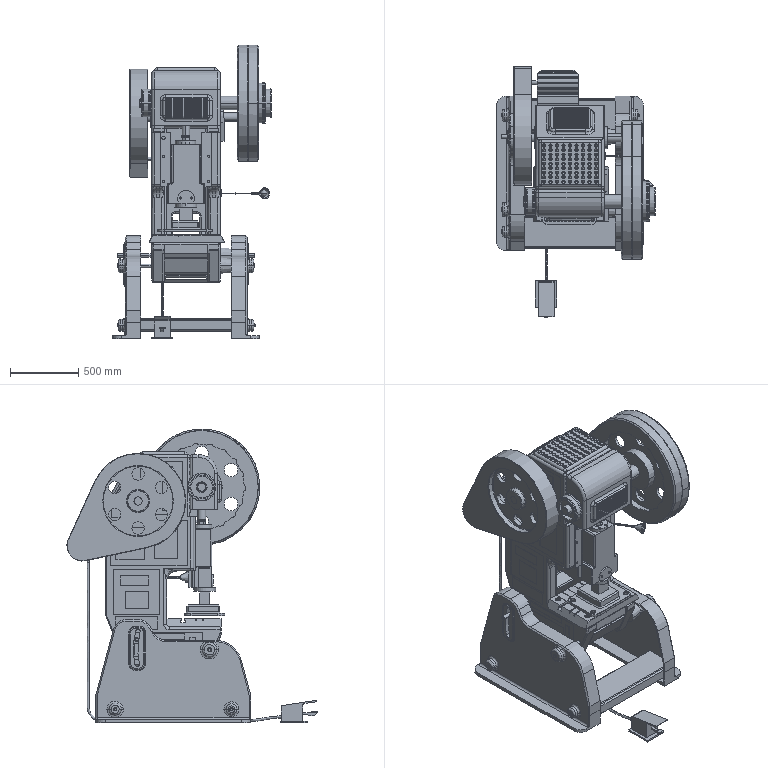Assembly | SolidWorks | mm | 53 component files | 53 solids | 4337 faces | box 1159 x 1828.89 x 2148.9 mm | volume 424193387 mm3 | plane 1614 | cylinder 1553 | cone 588 | spline 500 | torus 65 | sphere 17 | commonest cylinder face diameters 3.8 x373 21.383 x162 789.22 x156 20 x86 40 x68 10 x60 30 x44 61.909 x42
Bill of materials:
AxisHead | 1 |  | Short disc/wheel body with a shallow circumferential groove between two rim flanges, a smaller coaxial cylindrical boss with rounded edge on one face, and a shallow circular recess with a raised lip on the opposite face.
Belt | 3 |  | Thin closed loop shaped like a teardrop / rounded triangle: a large circular arc joined by two straight segments that meet at a small rounded corner. The section is very thin and the loop lies flat in one plane.
Cam | 1 |  | Rectangular block with rounded vertical edges and one large cylindrical through-hole passing through a pair of opposite side faces.
CamAxis | 1 |  | Plain solid cylindrical rod with flat ends.
ConnectingBeam | 2 |  | Elongated rectangular bar with angled chamfers at the end corners, light edge chamfers along the long edges, and a small coaxial cylindrical pin projecting from the centre of each end face. A small circular ring feature sits at the centre of one large face.
ConnectingBlock | 1 |  | Solid rectangular block with filleted or rounded edges on all sides. No holes or other features are visible.
ConnectingRod | 1 |  | Stepped turned pin: a cylindrical shank with a chamfered top and a narrow circumferential groove near its lower end, a hexagonal section below, and a two-step circular flange at the base.
CountersunkScrew | 6 |  | Countersunk (conical) flat-head fastener-like body with a cross-shaped recess in the head, a short reduced-diameter neck under the head, and a longer, larger-diameter cylindrical shank.
CylindricalHeadHexSocketScrew | 4 |  | Cylindrical head with a hexagonal socket on a plain, smaller-diameter cylindrical shank, similar in form to a socket head cap screw.
DriveShaft | 1 |  | Stepped cylinder: a larger-diameter main body with a small axial bore in one end face, and a smaller coaxial cylindrical pin projecting from the other end.
EndCapCover | 1 |  | Flanged circular cap: a thin round flange with six evenly spaced small holes around its edge, and a raised, closed cylindrical boss in the centre with a rounded top edge.
EndFacePressurePlate | 1 |  | Square flat plate of moderate thickness with seven through-holes of at least two diameters in an irregular pattern.
FixedAxis | 2 |  | Short prismatic body with an irregular five-sided, round-cornered cross-section, pierced axially by a straight slender cylindrical rod that sticks out a long way on both ends.
Flywheel | 1 |  | Thick annular ring (short hollow cylinder) with one central through bore and lightly rounded outer edges.
FootSwitch | 1 |  | Long thin wire or rod with a radiused bend, ending in a small box-shaped block with flanges and slots at one end.
Frame | 1 |  | Complex hollow housing or bracket body: a rectangular tube-like upper section with a square through opening, a ribbed raised pad on one face, a side profile with a C-shaped notch and angled lower edge, and an open lower frame.
Gland | 1 |  | Flat circular annular plate with a large central bore and six round through holes evenly spaced on a circle between bore and rim.
GuidePlate | 1 |  | Rectangular bar with a V-shaped groove along one long face and two small round through holes along its length.
LargeGear | 1 |  | Large spur-style gear with many fine straight teeth, a recessed web with six round lightening holes, and a protruding cylindrical hub on one side with a central bore.
LargePulley | 1 |  | Disk-shaped wheel with several circumferential grooves on its outer rim, a recessed face, six round holes on a circle, and a small central hole.
LeftBase | 1 |  | Flat profiled side plate with sloped sides and a raised rounded hump at one upper corner. It has a perimeter lip, a bottom flange along one edge, a curved arc-shaped slot with a raised boss around it, small holes, and cylindrical bosses on the back.
LeftGuideRail | 1 |  | Rectangular bar with a V-shaped groove along one long face and three small round through holes evenly spaced along its length.
Light | 1 |  | Circular disk base with a slender curved rod (S-bend) running to a conical cup-shaped head that holds a sphere.
Motor | 1 |  | Extruded block whose constant cross-section combines a large round lobe with many small radial fins, a rectangular tab with a C-shaped slot, and two rounded notches. It has longitudinal surface grooves, and a small stud with circumferential ribs on a narrow neck sticks out from one end face.
Pinion | 1 |  | Straight-toothed spur gear: a cylindrical body that is fairly wide relative to its diameter, with a central round bore that has one keyway notch.
Plate | 1 |  | Very thin, flat circular disc with no visible holes or features.
PressureBlock | 1 |  | Prismatic block with a rounded profile (circular-arc top and flat bottom), two through holes in the end face, and a semicircular cutout in one side.
PressureHead | 1 |  | Stepped pin-like part: a rectangular/square prism base, a thin circular flange above it with chamfered edges, and a smaller cylindrical pin sticking up from the flange center.
PressurePlate | 1 |  | Flat rectangular mounting plate with rounded corners, a raised rectangular boss with chamfered edges, and a square through opening in the center of the boss.
ProtectiveCover | 1 |  | Flat teardrop-shaped plate (round body tapering to a rounded point) with a large irregular inner opening whose edge has many small rounded notches, plus a small rectangular tab standing out from one face.
ProtectiveCoverII | 1 |  | Flat teardrop-shaped plate with a large irregular inner opening whose edge has many small rounded notches. It has no tab on its faces.
PulleyGuard | 1 |  | Teardrop-shaped flat plate of uniform thickness with one large circular through hole placed concentric with the rounded end.
RightBase | 1 |  | Plate-like bracket with an irregular stepped top outline, a narrow curved slot, three raised round bosses with small holes, and a thin lip or foot running along the bottom edge.
Screw | 1 |  | Hex-head bolt-like part with a plain cylindrical shank.
Slider | 1 |  | Block-shaped body with a tall rectangular upper section ending in angled or dovetail-like side projections, a wider lower section with side shoulders, and a half-cylinder channel with two small holes at the lower end.
SpacerBlock | 2 |  | Truncated cone (frustum) with a central through bore along its axis.
SpindleBody | 1 |  | Straight solid cylindrical rod with flat, square-cut ends; long and slender.
TopPlate | 1 |  | Thin rectangular plate with rounded corners and rounded perimeter edges, carrying a regular 9 x 9 grid of circular, conical-bottomed recesses on one face.
UpperHousing | 1 |  | Compact block with a D-shaped profile: one flat side, a quarter-round rounded top along its length, a single round through-hole crossing the end faces, and a raised rectangular pad with fine parallel ribs on one long face.
WorkbenchPanel | 1 |  | Flat rectangular plate with bevelled long edges, a large central circular through-hole, four small corner holes, a pattern of shallow parallel grooves across the top face, one deeper lengthwise slot, and small notches/slots along the edges.
Mates:
1. coincident | RightBase-1 face at (-30.67, 577.837, -607.551) dir (0, 0, -1) | FootSwitch-2 face at (-755.332, 295.499, -607.551) dir (0, 0, -1)
2. distance | FootSwitch-2 face at (-598.332, -254.638, -1191.775) dir (1, 0, 0) | RightBase-1 face at (-171.332, 1419.395, 47.449) dir (-1, 0, 0)
3. distance | FootSwitch-2 face at (-755.332, 295.499, -595.551) dir (0, 1, 0) | RightBase-1 face at (-72.332, 513.499, -553.551) dir (0, -1, 0)
4. coincident | Frame-1 face at (-254.332, 1221.845, -37.038) dir (1, 0, 0) | Light-1 face at (-254.332, 1202.548, 457.059) dir (-1, 0, 0)
5. distance | Light-1 face at (-241.332, 1202.548, 457.059) dir (-1, 0, 0) r 25 | Frame-1 face at (-252.332, 1127.548, 423.663) dir (0, -1, 0)